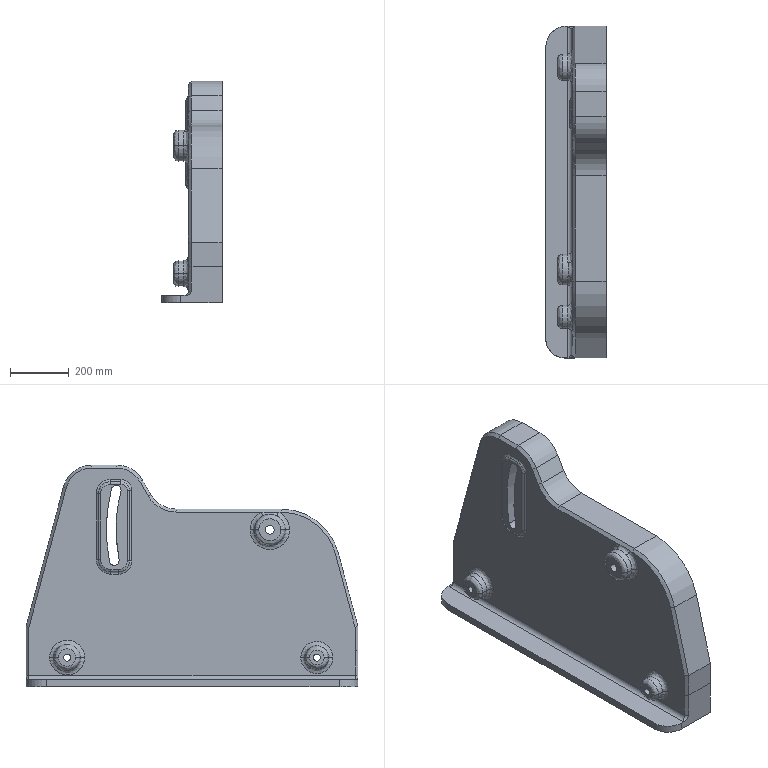Component | SolidWorks | LeftBase-1 | 1 solid | 141 faces | volume 21151507 mm3 | cylinder 47 | plane 45 | cone 27 | spline 22 | commonest cylinder face diameters 20 x8 30 x5 24 x4 57 x4 33 x4 200 x3 83.378 x2 79.335 x2